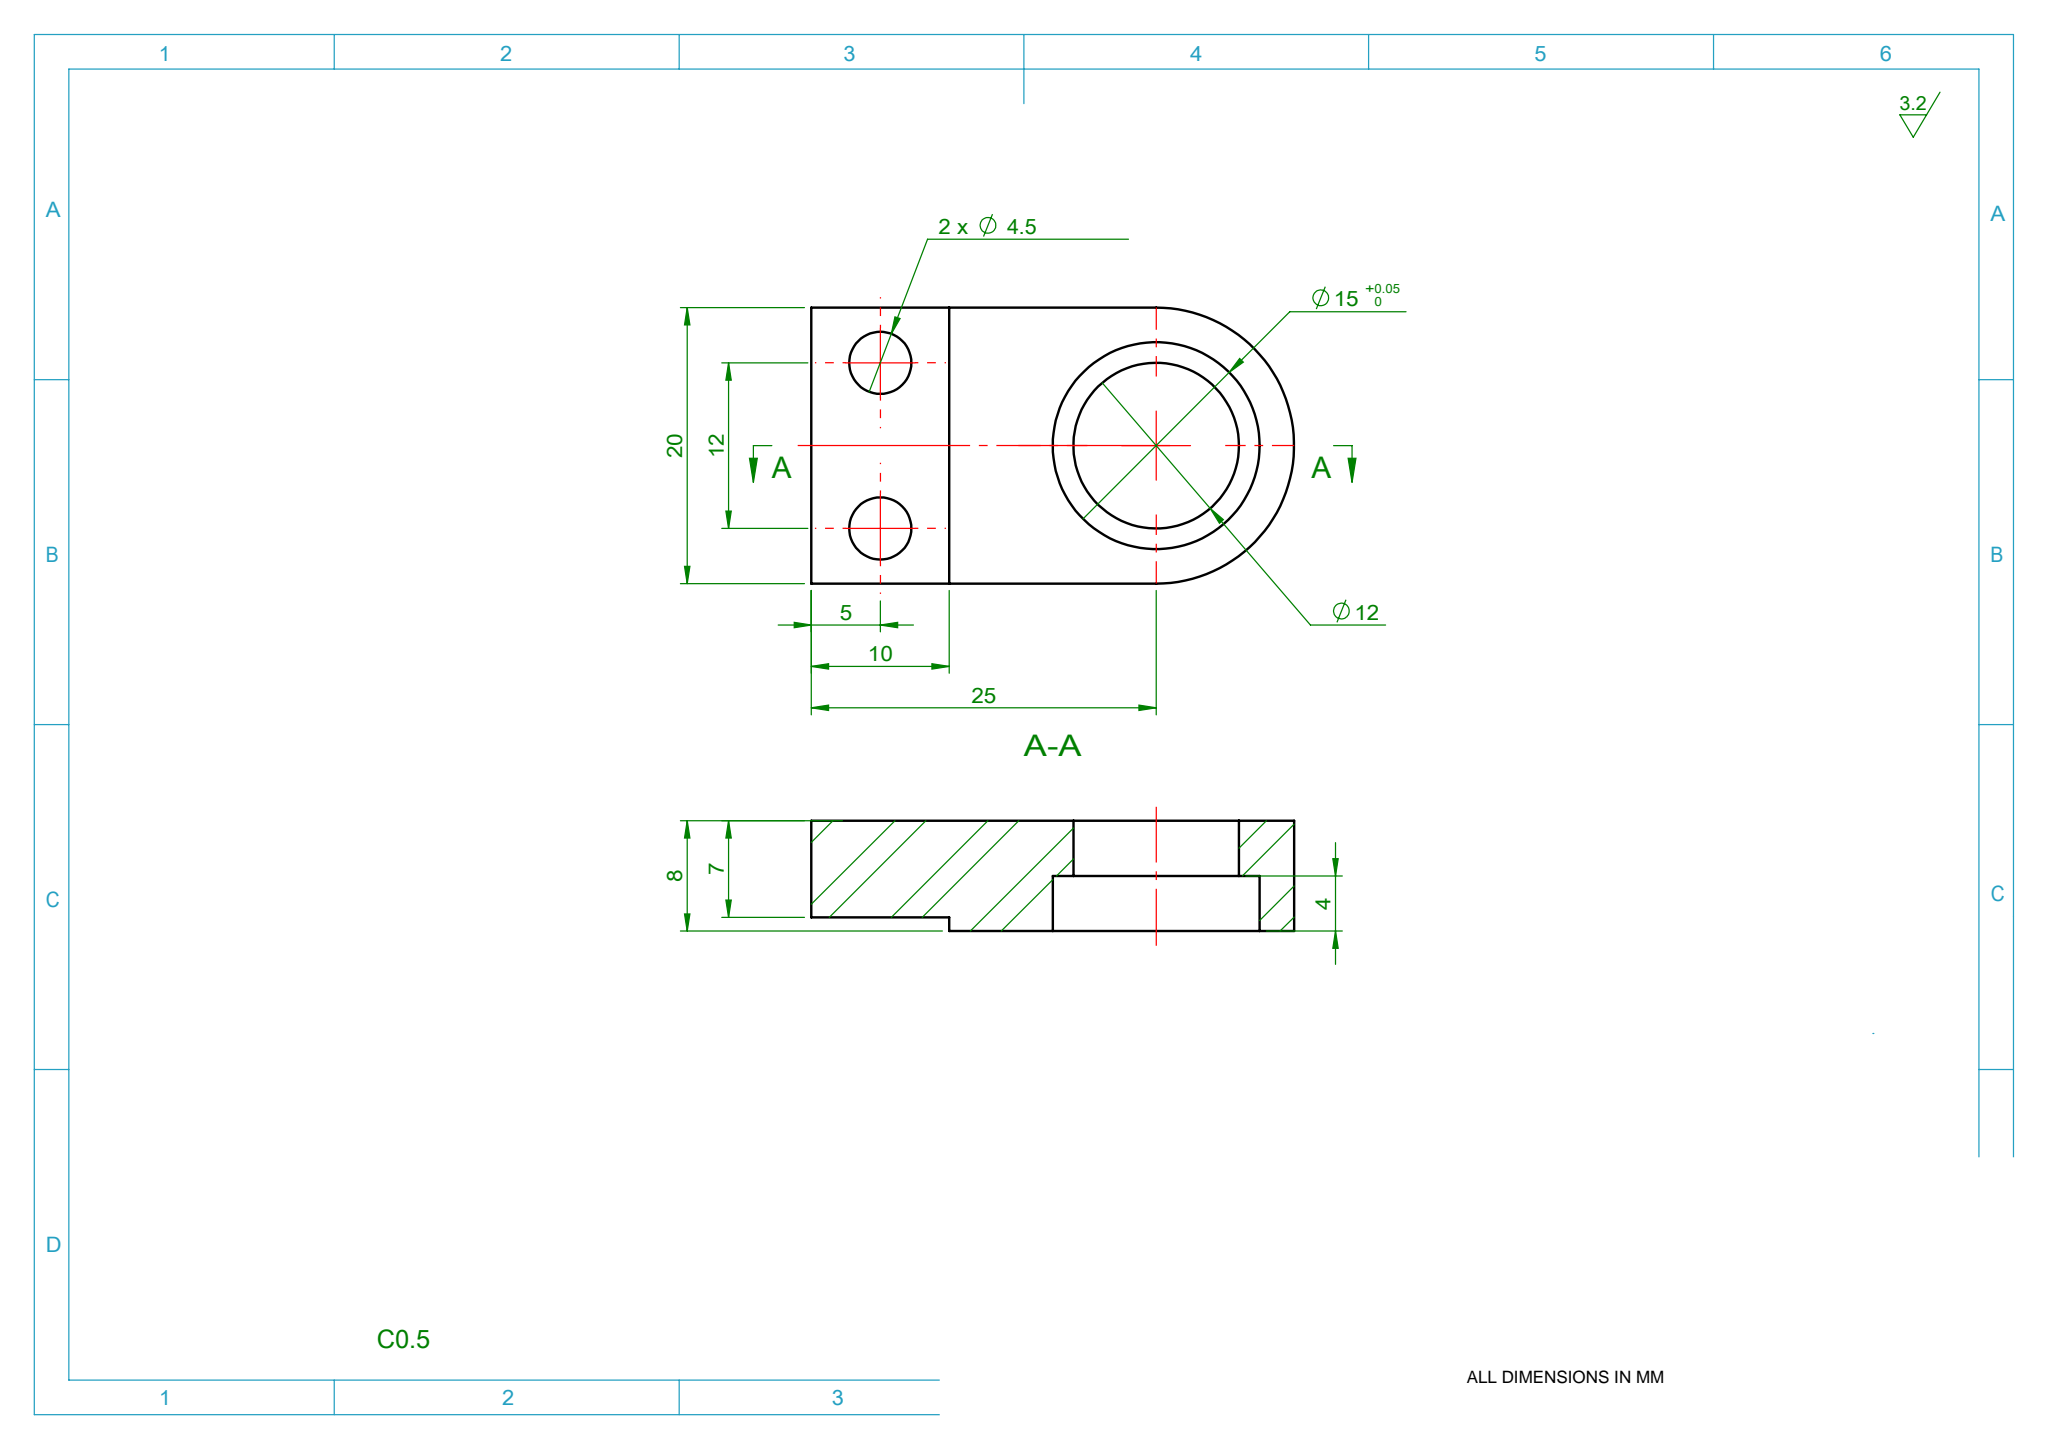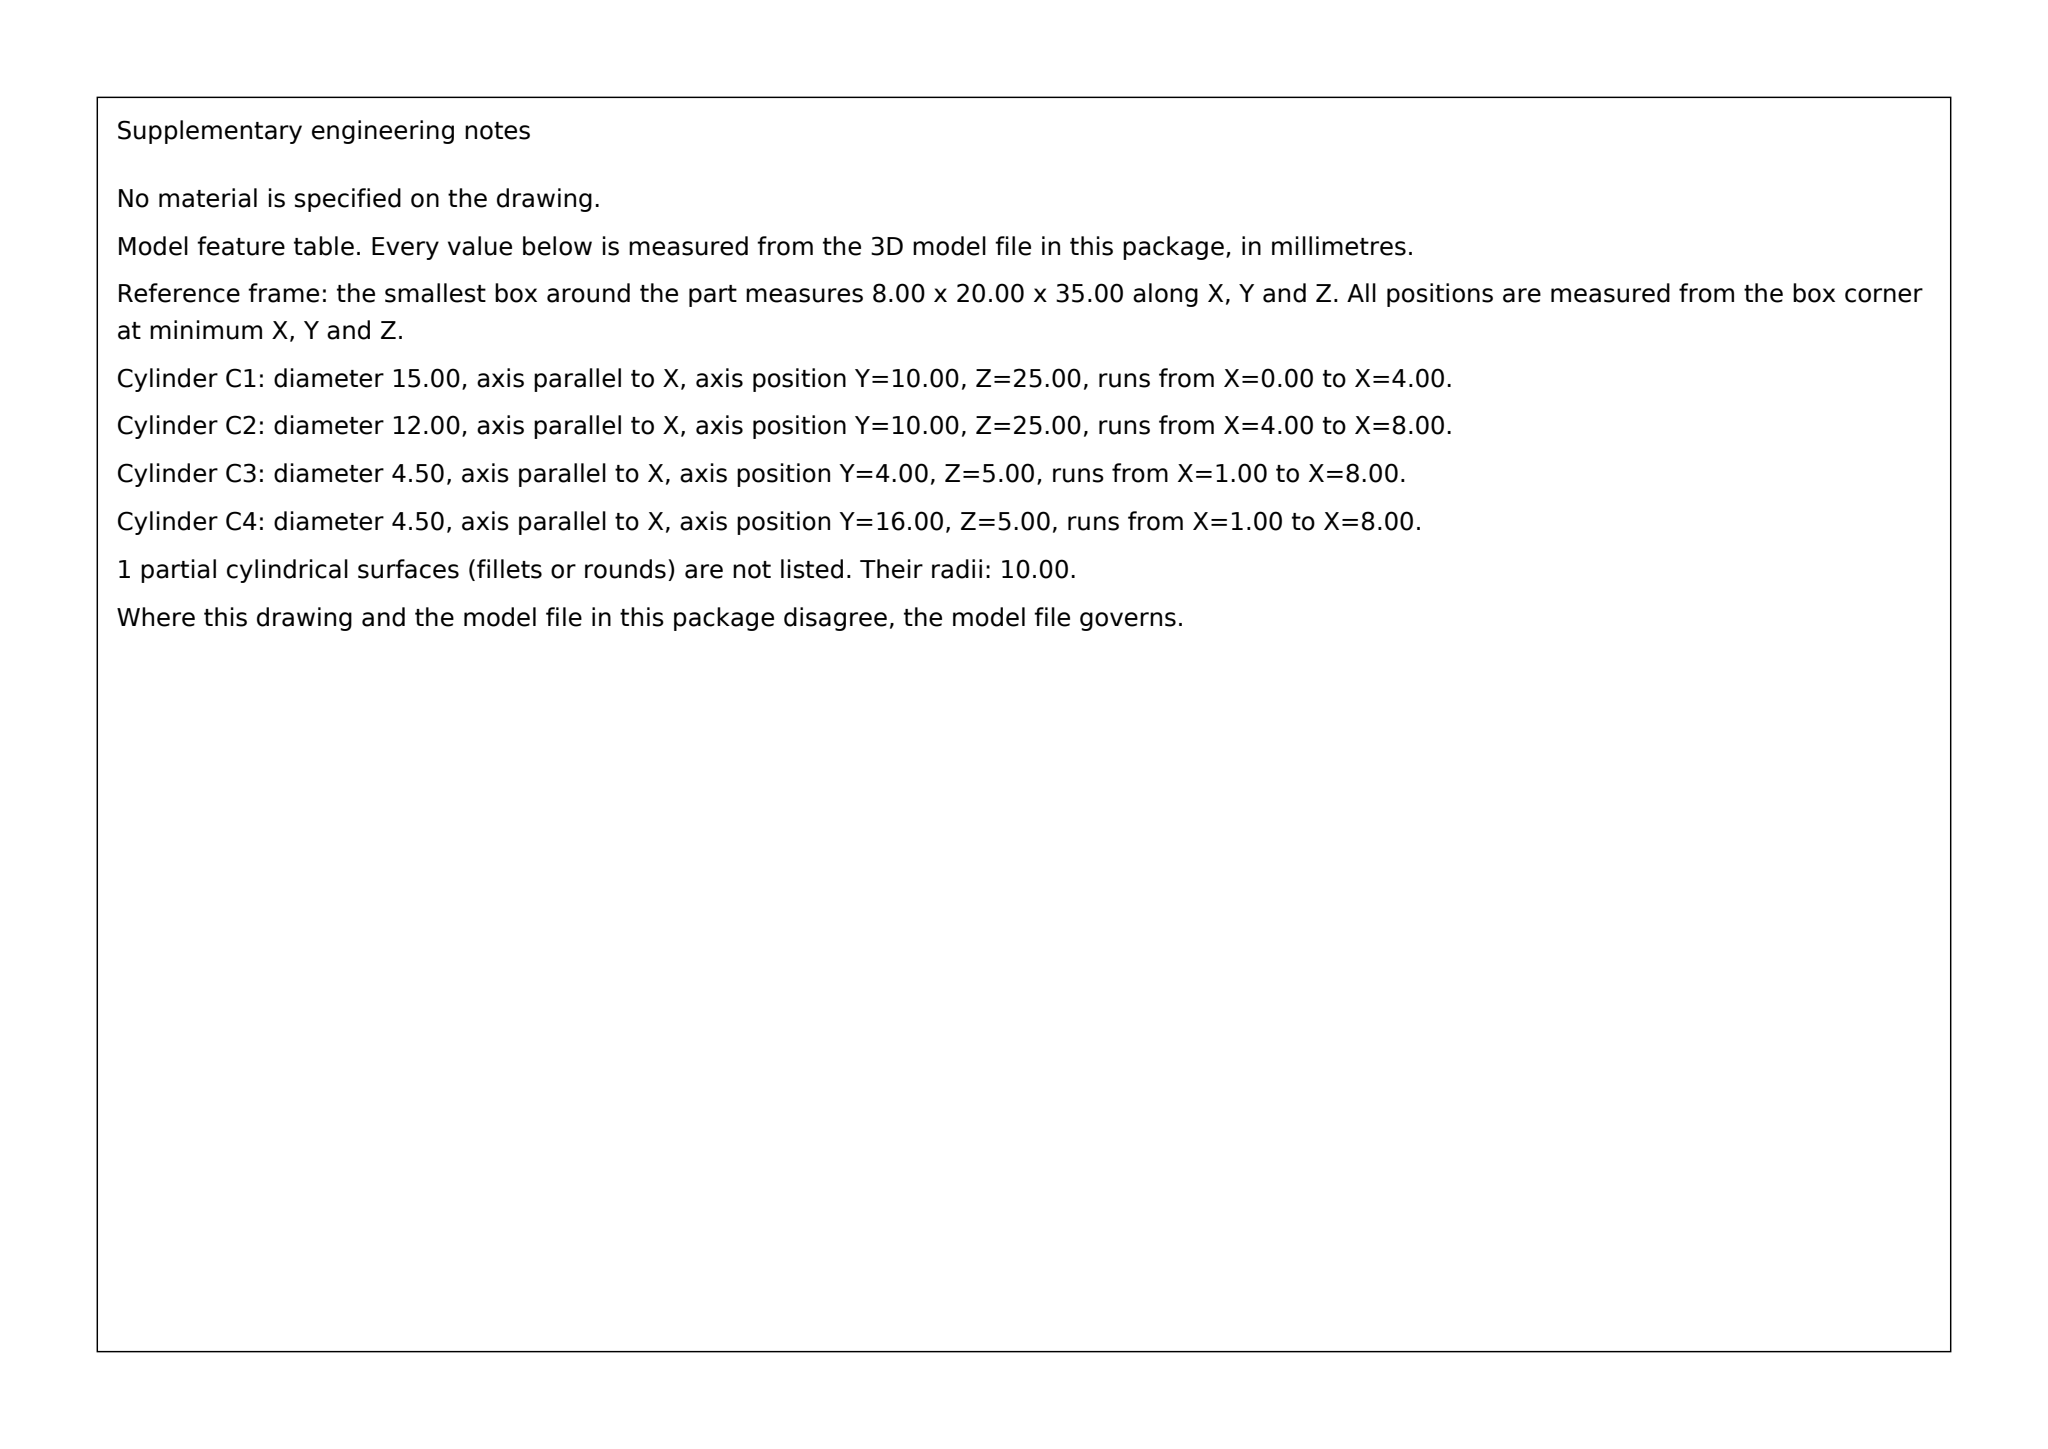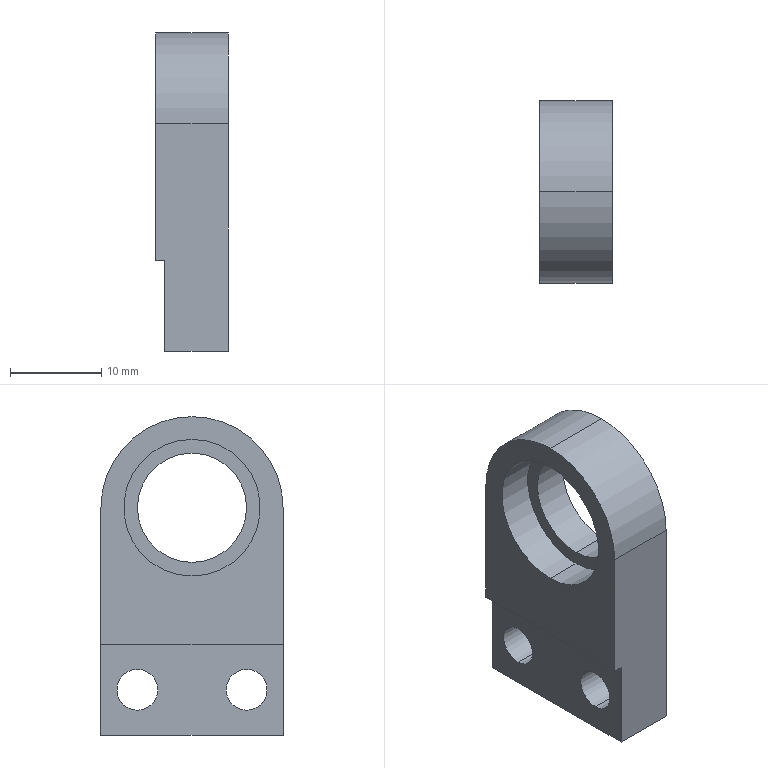Part | SolidWorks | mm | 1 solid | 18 faces | box 8 x 20 x 35 mm | volume 3675 mm3 | cylinder 10 | plane 8 | commonest cylinder face diameters 4.5 x4 12 x2 15 x2 20 x2
build123d program:
from build123d import *

# Parameters (mm, degrees)
BOSS_EXTRUDE1_DEPTH  = 8
SKETCH2_R            = 7.5
CUT_EXTRUDE1_DEPTH   = 4
SKETCH3_R            = 6
CUT_EXTRUDE2_DEPTH   = 28.221
SKETCH4_W            = 10
SKETCH4_H            = 20
CUT_EXTRUDE3_DEPTH   = 1
M4_CLEARANCE_HOLE1_D = 4.5


with BuildPart() as part:
    # Sketch1 → Boss-Extrude1 (new body)
    with BuildSketch(Plane(origin=(0, 0, 0), x_dir=(0, 0, -1), z_dir=(1, 0, 0))):
        with BuildLine():
            Line((0, 10), (25, 10))
            Line((25, 10), (25, -10))
            Line((25, -10), (0, -10))
            ThreePointArc((0, -10), (-10, 0), (0, 10))
        make_face()
    extrude(amount=BOSS_EXTRUDE1_DEPTH)

    # Sketch2 → Cut-Extrude1 (cut)
    with BuildSketch(Plane.ZY):
        Circle(SKETCH2_R)
    extrude(amount=-CUT_EXTRUDE1_DEPTH, mode=Mode.SUBTRACT)

    # Sketch3 → Cut-Extrude2 (cut, through all)
    with BuildSketch(Plane.ZY.offset(-4)):
        Circle(SKETCH3_R)
    extrude(amount=-CUT_EXTRUDE2_DEPTH, mode=Mode.SUBTRACT)

    # Sketch4 → Cut-Extrude3 (cut)
    with BuildSketch(Plane.ZY):
        with Locations((-20, 0)):
            Rectangle(SKETCH4_W, SKETCH4_H)
    extrude(amount=-CUT_EXTRUDE3_DEPTH, mode=Mode.SUBTRACT)

    # M4 Clearance Hole1 (through all)
    with Locations(Plane(origin=(8, 0, 0), x_dir=(0, 0, -1), z_dir=(1, 0, 0))):
        with Locations((20, 6), (20, -6)):
            Hole(M4_CLEARANCE_HOLE1_D / 2)


solid = part.part
STEP:
#1=CARTESIAN_POINT('',(1.,6.,-22.25));
#2=VERTEX_POINT('',#1);
#3=CARTESIAN_POINT('',(1.,6.,-17.75));
#4=VERTEX_POINT('',#3);
#5=CARTESIAN_POINT('',(1.,6.,-20.));
#6=DIRECTION('',(-1.,0.,0.));
#7=DIRECTION('',(0.,0.,1.));
#8=AXIS2_PLACEMENT_3D('',#5,#6,#7);
#9=CIRCLE('',#8,2.25);
#10=EDGE_CURVE('',#2,#4,#9,.T.);
#11=ORIENTED_EDGE('',*,*,#10,.T.);
#12=CARTESIAN_POINT('',(8.,6.,-17.75));
#13=VERTEX_POINT('',#12);
#14=CARTESIAN_POINT('',(8.,6.,-17.75));
#15=DIRECTION('',(1.,0.,0.));
#16=VECTOR('',#15,1000.);
#17=LINE('',#14,#16);
#18=EDGE_CURVE('',#4,#13,#17,.T.);
#19=ORIENTED_EDGE('',*,*,#18,.T.);
#20=CARTESIAN_POINT('',(8.,6.,-22.25));
#21=VERTEX_POINT('',#20);
#22=CARTESIAN_POINT('',(8.,6.,-20.));
#23=DIRECTION('',(1.,0.,0.));
#24=DIRECTION('',(0.,0.,-1.));
#25=AXIS2_PLACEMENT_3D('',#22,#23,#24);
#26=CIRCLE('',#25,2.25);
#27=EDGE_CURVE('',#13,#21,#26,.T.);
#28=ORIENTED_EDGE('',*,*,#27,.T.);
#29=CARTESIAN_POINT('',(8.,6.,-22.25));
#30=DIRECTION('',(1.,0.,0.));
#31=VECTOR('',#30,1000.);
#32=LINE('',#29,#31);
#33=EDGE_CURVE('',#2,#21,#32,.T.);
#34=ORIENTED_EDGE('',*,*,#33,.F.);
#35=EDGE_LOOP('',(#11,#19,#28,#34));
#36=FACE_OUTER_BOUND('',#35,.T.);
#37=CARTESIAN_POINT('',(8.,6.,-20.));
#38=DIRECTION('',(1.,0.,0.));
#39=DIRECTION('',(0.,0.,-1.));
#40=AXIS2_PLACEMENT_3D('',#37,#38,#39);
#41=CYLINDRICAL_SURFACE('',#40,2.25);
#42=ADVANCED_FACE('',(#36),#41,.F.);
#43=CARTESIAN_POINT('',(1.,-6.,-22.25));
#44=VERTEX_POINT('',#43);
#45=CARTESIAN_POINT('',(1.,-6.,-17.75));
#46=VERTEX_POINT('',#45);
#47=CARTESIAN_POINT('',(1.,-6.,-20.));
#48=DIRECTION('',(-1.,0.,0.));
#49=DIRECTION('',(0.,0.,1.));
#50=AXIS2_PLACEMENT_3D('',#47,#48,#49);
#51=CIRCLE('',#50,2.25);
#52=EDGE_CURVE('',#44,#46,#51,.T.);
#53=ORIENTED_EDGE('',*,*,#52,.T.);
#54=CARTESIAN_POINT('',(8.,-6.,-17.75));
#55=VERTEX_POINT('',#54);
#56=CARTESIAN_POINT('',(8.,-6.,-17.75));
#57=DIRECTION('',(1.,0.,0.));
#58=VECTOR('',#57,1000.);
#59=LINE('',#56,#58);
#60=EDGE_CURVE('',#46,#55,#59,.T.);
#61=ORIENTED_EDGE('',*,*,#60,.T.);
#62=CARTESIAN_POINT('',(8.,-6.,-22.25));
#63=VERTEX_POINT('',#62);
#64=CARTESIAN_POINT('',(8.,-6.,-20.));
#65=DIRECTION('',(1.,0.,0.));
#66=DIRECTION('',(0.,0.,-1.));
#67=AXIS2_PLACEMENT_3D('',#64,#65,#66);
#68=CIRCLE('',#67,2.25);
#69=EDGE_CURVE('',#55,#63,#68,.T.);
#70=ORIENTED_EDGE('',*,*,#69,.T.);
#71=CARTESIAN_POINT('',(8.,-6.,-22.25));
#72=DIRECTION('',(1.,0.,0.));
#73=VECTOR('',#72,1000.);
#74=LINE('',#71,#73);
#75=EDGE_CURVE('',#44,#63,#74,.T.);
#76=ORIENTED_EDGE('',*,*,#75,.F.);
#77=EDGE_LOOP('',(#53,#61,#70,#76));
#78=FACE_OUTER_BOUND('',#77,.T.);
#79=CARTESIAN_POINT('',(8.,-6.,-20.));
#80=DIRECTION('',(1.,0.,0.));
#81=DIRECTION('',(0.,0.,-1.));
#82=AXIS2_PLACEMENT_3D('',#79,#80,#81);
#83=CYLINDRICAL_SURFACE('',#82,2.25);
#84=ADVANCED_FACE('',(#78),#83,.F.);
#85=CARTESIAN_POINT('',(8.,0.,-6.));
#86=VERTEX_POINT('',#85);
#87=CARTESIAN_POINT('',(8.,0.,6.));
#88=VERTEX_POINT('',#87);
#89=CARTESIAN_POINT('',(8.,0.,0.));
#90=DIRECTION('',(-1.,0.,0.));
#91=DIRECTION('',(0.,0.,1.));
#92=AXIS2_PLACEMENT_3D('',#89,#90,#91);
#93=CIRCLE('',#92,6.);
#94=EDGE_CURVE('',#86,#88,#93,.T.);
#95=ORIENTED_EDGE('',*,*,#94,.F.);
#96=CARTESIAN_POINT('',(4.,0.,-6.));
#97=VERTEX_POINT('',#96);
#98=CARTESIAN_POINT('',(8.,0.,-6.));
#99=DIRECTION('',(-1.,0.,0.));
#100=VECTOR('',#99,1000.);
#101=LINE('',#98,#100);
#102=EDGE_CURVE('',#86,#97,#101,.T.);
#103=ORIENTED_EDGE('',*,*,#102,.T.);
#104=CARTESIAN_POINT('',(4.,0.,6.));
#105=VERTEX_POINT('',#104);
#106=CARTESIAN_POINT('',(4.,0.,0.));
#107=DIRECTION('',(-1.,0.,0.));
#108=DIRECTION('',(0.,0.,1.));
#109=AXIS2_PLACEMENT_3D('',#106,#107,#108);
#110=CIRCLE('',#109,6.);
#111=EDGE_CURVE('',#97,#105,#110,.T.);
#112=ORIENTED_EDGE('',*,*,#111,.T.);
#113=CARTESIAN_POINT('',(8.,0.,6.));
#114=DIRECTION('',(-1.,0.,0.));
#115=VECTOR('',#114,1000.);
#116=LINE('',#113,#115);
#117=EDGE_CURVE('',#88,#105,#116,.T.);
#118=ORIENTED_EDGE('',*,*,#117,.F.);
#119=EDGE_LOOP('',(#95,#103,#112,#118));
#120=FACE_OUTER_BOUND('',#119,.T.);
#121=CARTESIAN_POINT('',(8.,0.,0.));
#122=DIRECTION('',(-1.,0.,0.));
#123=DIRECTION('',(0.,0.,1.));
#124=AXIS2_PLACEMENT_3D('',#121,#122,#123);
#125=CYLINDRICAL_SURFACE('',#124,6.);
#126=ADVANCED_FACE('',(#120),#125,.F.);
#127=CARTESIAN_POINT('',(4.,0.,-7.5));
#128=VERTEX_POINT('',#127);
#129=CARTESIAN_POINT('',(4.,0.,7.5));
#130=VERTEX_POINT('',#129);
#131=CARTESIAN_POINT('',(4.,0.,0.));
#132=DIRECTION('',(-1.,0.,0.));
#133=DIRECTION('',(0.,0.,1.));
#134=AXIS2_PLACEMENT_3D('',#131,#132,#133);
#135=CIRCLE('',#134,7.5);
#136=EDGE_CURVE('',#128,#130,#135,.T.);
#137=ORIENTED_EDGE('',*,*,#136,.F.);
#138=CARTESIAN_POINT('',(0.,0.,-7.5));
#139=VERTEX_POINT('',#138);
#140=CARTESIAN_POINT('',(4.,0.,-7.5));
#141=DIRECTION('',(-1.,0.,0.));
#142=VECTOR('',#141,1000.);
#143=LINE('',#140,#142);
#144=EDGE_CURVE('',#128,#139,#143,.T.);
#145=ORIENTED_EDGE('',*,*,#144,.T.);
#146=CARTESIAN_POINT('',(0.,0.,7.5));
#147=VERTEX_POINT('',#146);
#148=CARTESIAN_POINT('',(0.,0.,0.));
#149=DIRECTION('',(-1.,0.,0.));
#150=DIRECTION('',(0.,0.,1.));
#151=AXIS2_PLACEMENT_3D('',#148,#149,#150);
#152=CIRCLE('',#151,7.5);
#153=EDGE_CURVE('',#139,#147,#152,.T.);
#154=ORIENTED_EDGE('',*,*,#153,.T.);
#155=CARTESIAN_POINT('',(4.,0.,7.5));
#156=DIRECTION('',(-1.,0.,0.));
#157=VECTOR('',#156,1000.);
#158=LINE('',#155,#157);
#159=EDGE_CURVE('',#130,#147,#158,.T.);
#160=ORIENTED_EDGE('',*,*,#159,.F.);
#161=EDGE_LOOP('',(#137,#145,#154,#160));
#162=FACE_OUTER_BOUND('',#161,.T.);
#163=CARTESIAN_POINT('',(4.,0.,0.));
#164=DIRECTION('',(-1.,0.,0.));
#165=DIRECTION('',(0.,0.,1.));
#166=AXIS2_PLACEMENT_3D('',#163,#164,#165);
#167=CYLINDRICAL_SURFACE('',#166,7.5);
#168=ADVANCED_FACE('',(#162),#167,.F.);
#169=CARTESIAN_POINT('',(8.,0.,10.));
#170=VERTEX_POINT('',#169);
#171=CARTESIAN_POINT('',(8.,-10.,0.));
#172=VERTEX_POINT('',#171);
#173=CARTESIAN_POINT('',(8.,0.,0.));
#174=DIRECTION('',(1.,0.,0.));
#175=DIRECTION('',(0.,0.,-1.));
#176=AXIS2_PLACEMENT_3D('',#173,#174,#175);
#177=CIRCLE('',#176,10.);
#178=EDGE_CURVE('',#170,#172,#177,.T.);
#179=ORIENTED_EDGE('',*,*,#178,.F.);
#180=CARTESIAN_POINT('',(0.,0.,10.));
#181=VERTEX_POINT('',#180);
#182=CARTESIAN_POINT('',(8.,0.,10.));
#183=DIRECTION('',(-1.,0.,0.));
#184=VECTOR('',#183,1000.);
#185=LINE('',#182,#184);
#186=EDGE_CURVE('',#170,#181,#185,.T.);
#187=ORIENTED_EDGE('',*,*,#186,.T.);
#188=CARTESIAN_POINT('',(0.,-10.,0.));
#189=VERTEX_POINT('',#188);
#190=CARTESIAN_POINT('',(0.,0.,0.));
#191=DIRECTION('',(1.,0.,0.));
#192=DIRECTION('',(0.,0.,-1.));
#193=AXIS2_PLACEMENT_3D('',#190,#191,#192);
#194=CIRCLE('',#193,10.);
#195=EDGE_CURVE('',#181,#189,#194,.T.);
#196=ORIENTED_EDGE('',*,*,#195,.T.);
#197=CARTESIAN_POINT('',(8.,-10.,0.));
#198=DIRECTION('',(-1.,0.,0.));
#199=VECTOR('',#198,1000.);
#200=LINE('',#197,#199);
#201=EDGE_CURVE('',#172,#189,#200,.T.);
#202=ORIENTED_EDGE('',*,*,#201,.F.);
#203=EDGE_LOOP('',(#179,#187,#196,#202));
#204=FACE_OUTER_BOUND('',#203,.T.);
#205=CARTESIAN_POINT('',(8.,0.,0.));
#206=DIRECTION('',(-1.,0.,0.));
#207=DIRECTION('',(0.,0.,1.));
#208=AXIS2_PLACEMENT_3D('',#205,#206,#207);
#209=CYLINDRICAL_SURFACE('',#208,10.);
#210=ADVANCED_FACE('',(#204),#209,.T.);
#211=CARTESIAN_POINT('',(1.,10.,-25.));
#212=VERTEX_POINT('',#211);
#213=CARTESIAN_POINT('',(1.,-10.,-25.));
#214=VERTEX_POINT('',#213);
#215=CARTESIAN_POINT('',(1.,-10.,-25.));
#216=DIRECTION('',(0.,-1.,0.));
#217=VECTOR('',#216,1000.);
#218=LINE('',#215,#217);
#219=EDGE_CURVE('',#212,#214,#218,.T.);
#220=ORIENTED_EDGE('',*,*,#219,.F.);
#221=CARTESIAN_POINT('',(8.,10.,-25.));
#222=VERTEX_POINT('',#221);
#223=CARTESIAN_POINT('',(8.,10.,-25.));
#224=DIRECTION('',(-1.,0.,0.));
#225=VECTOR('',#224,1000.);
#226=LINE('',#223,#225);
#227=EDGE_CURVE('',#222,#212,#226,.T.);
#228=ORIENTED_EDGE('',*,*,#227,.F.);
#229=CARTESIAN_POINT('',(8.,-10.,-25.));
#230=VERTEX_POINT('',#229);
#231=CARTESIAN_POINT('',(8.,10.,-25.));
#232=DIRECTION('',(0.,1.,0.));
#233=VECTOR('',#232,1000.);
#234=LINE('',#231,#233);
#235=EDGE_CURVE('',#230,#222,#234,.T.);
#236=ORIENTED_EDGE('',*,*,#235,.F.);
#237=CARTESIAN_POINT('',(8.,-10.,-25.));
#238=DIRECTION('',(-1.,0.,0.));
#239=VECTOR('',#238,1000.);
#240=LINE('',#237,#239);
#241=EDGE_CURVE('',#230,#214,#240,.T.);
#242=ORIENTED_EDGE('',*,*,#241,.T.);
#243=EDGE_LOOP('',(#220,#228,#236,#242));
#244=FACE_OUTER_BOUND('',#243,.T.);
#245=CARTESIAN_POINT('',(8.,10.,-25.));
#246=DIRECTION('',(0.,0.,1.));
#247=DIRECTION('',(1.,0.,0.));
#248=AXIS2_PLACEMENT_3D('',#245,#246,#247);
#249=PLANE('',#248);
#250=ADVANCED_FACE('',(#244),#249,.F.);
#251=ORIENTED_EDGE('',*,*,#186,.F.);
#252=CARTESIAN_POINT('',(8.,10.,0.));
#253=VERTEX_POINT('',#252);
#254=CARTESIAN_POINT('',(8.,0.,0.));
#255=DIRECTION('',(1.,0.,0.));
#256=DIRECTION('',(0.,0.,-1.));
#257=AXIS2_PLACEMENT_3D('',#254,#255,#256);
#258=CIRCLE('',#257,10.);
#259=EDGE_CURVE('',#253,#170,#258,.T.);
#260=ORIENTED_EDGE('',*,*,#259,.F.);
#261=CARTESIAN_POINT('',(0.,10.,0.));
#262=VERTEX_POINT('',#261);
#263=CARTESIAN_POINT('',(8.,10.,0.));
#264=DIRECTION('',(-1.,0.,0.));
#265=VECTOR('',#264,1000.);
#266=LINE('',#263,#265);
#267=EDGE_CURVE('',#253,#262,#266,.T.);
#268=ORIENTED_EDGE('',*,*,#267,.T.);
#269=CARTESIAN_POINT('',(0.,0.,0.));
#270=DIRECTION('',(1.,0.,0.));
#271=DIRECTION('',(0.,0.,-1.));
#272=AXIS2_PLACEMENT_3D('',#269,#270,#271);
#273=CIRCLE('',#272,10.);
#274=EDGE_CURVE('',#262,#181,#273,.T.);
#275=ORIENTED_EDGE('',*,*,#274,.T.);
#276=EDGE_LOOP('',(#251,#260,#268,#275));
#277=FACE_OUTER_BOUND('',#276,.T.);
#278=CARTESIAN_POINT('',(8.,0.,0.));
#279=DIRECTION('',(-1.,0.,0.));
#280=DIRECTION('',(0.,0.,1.));
#281=AXIS2_PLACEMENT_3D('',#278,#279,#280);
#282=CYLINDRICAL_SURFACE('',#281,10.);
#283=ADVANCED_FACE('',(#277),#282,.T.);
#284=CARTESIAN_POINT('',(0.,-10.,-15.));
#285=VERTEX_POINT('',#284);
#286=CARTESIAN_POINT('',(0.,-10.,0.));
#287=DIRECTION('',(0.,0.,-1.));
#288=VECTOR('',#287,1000.);
#289=LINE('',#286,#288);
#290=EDGE_CURVE('',#189,#285,#289,.T.);
#291=ORIENTED_EDGE('',*,*,#290,.T.);
#292=CARTESIAN_POINT('',(1.,-10.,-15.));
#293=VERTEX_POINT('',#292);
#294=CARTESIAN_POINT('',(1.,-10.,-15.));
#295=DIRECTION('',(-1.,0.,0.));
#296=VECTOR('',#295,1000.);
#297=LINE('',#294,#296);
#298=EDGE_CURVE('',#293,#285,#297,.T.);
#299=ORIENTED_EDGE('',*,*,#298,.F.);
#300=CARTESIAN_POINT('',(1.,-10.,-15.));
#301=DIRECTION('',(0.,0.,1.));
#302=VECTOR('',#301,1000.);
#303=LINE('',#300,#302);
#304=EDGE_CURVE('',#214,#293,#303,.T.);
#305=ORIENTED_EDGE('',*,*,#304,.F.);
#306=ORIENTED_EDGE('',*,*,#241,.F.);
#307=CARTESIAN_POINT('',(8.,-10.,0.));
#308=DIRECTION('',(0.,0.,-1.));
#309=VECTOR('',#308,1000.);
#310=LINE('',#307,#309);
#311=EDGE_CURVE('',#172,#230,#310,.T.);
#312=ORIENTED_EDGE('',*,*,#311,.F.);
#313=ORIENTED_EDGE('',*,*,#201,.T.);
#314=EDGE_LOOP('',(#291,#299,#305,#306,#312,#313));
#315=FACE_OUTER_BOUND('',#314,.T.);
#316=CARTESIAN_POINT('',(8.,-10.,0.));
#317=DIRECTION('',(0.,1.,0.));
#318=DIRECTION('',(0.,0.,1.));
#319=AXIS2_PLACEMENT_3D('',#316,#317,#318);
#320=PLANE('',#319);
#321=ADVANCED_FACE('',(#315),#320,.F.);
#322=CARTESIAN_POINT('',(1.,10.,-15.));
#323=VERTEX_POINT('',#322);
#324=CARTESIAN_POINT('',(1.,10.,-15.));
#325=DIRECTION('',(0.,0.,-1.));
#326=VECTOR('',#325,1000.);
#327=LINE('',#324,#326);
#328=EDGE_CURVE('',#323,#212,#327,.T.);
#329=ORIENTED_EDGE('',*,*,#328,.F.);
#330=CARTESIAN_POINT('',(0.,10.,-15.));
#331=VERTEX_POINT('',#330);
#332=CARTESIAN_POINT('',(1.,10.,-15.));
#333=DIRECTION('',(-1.,0.,0.));
#334=VECTOR('',#333,1000.);
#335=LINE('',#332,#334);
#336=EDGE_CURVE('',#323,#331,#335,.T.);
#337=ORIENTED_EDGE('',*,*,#336,.T.);
#338=CARTESIAN_POINT('',(0.,10.,0.));
#339=DIRECTION('',(0.,0.,1.));
#340=VECTOR('',#339,1000.);
#341=LINE('',#338,#340);
#342=EDGE_CURVE('',#331,#262,#341,.T.);
#343=ORIENTED_EDGE('',*,*,#342,.T.);
#344=ORIENTED_EDGE('',*,*,#267,.F.);
#345=CARTESIAN_POINT('',(8.,10.,0.));
#346=DIRECTION('',(0.,0.,1.));
#347=VECTOR('',#346,1000.);
#348=LINE('',#345,#347);
#349=EDGE_CURVE('',#222,#253,#348,.T.);
#350=ORIENTED_EDGE('',*,*,#349,.F.);
#351=ORIENTED_EDGE('',*,*,#227,.T.);
#352=EDGE_LOOP('',(#329,#337,#343,#344,#350,#351));
#353=FACE_OUTER_BOUND('',#352,.T.);
#354=CARTESIAN_POINT('',(8.,10.,0.));
#355=DIRECTION('',(0.,-1.,0.));
#356=DIRECTION('',(0.,0.,-1.));
#357=AXIS2_PLACEMENT_3D('',#354,#355,#356);
#358=PLANE('',#357);
#359=ADVANCED_FACE('',(#353),#358,.F.);
#360=CARTESIAN_POINT('',(8.,6.,-20.));
#361=DIRECTION('',(1.,0.,0.));
#362=DIRECTION('',(0.,0.,-1.));
#363=AXIS2_PLACEMENT_3D('',#360,#361,#362);
#364=CIRCLE('',#363,2.25);
#365=EDGE_CURVE('',#21,#13,#364,.T.);
#366=ORIENTED_EDGE('',*,*,#365,.F.);
#367=ORIENTED_EDGE('',*,*,#27,.F.);
#368=EDGE_LOOP('',(#366,#367));
#369=FACE_BOUND('',#368,.T.);
#370=CARTESIAN_POINT('',(8.,-6.,-20.));
#371=DIRECTION('',(1.,0.,0.));
#372=DIRECTION('',(0.,0.,-1.));
#373=AXIS2_PLACEMENT_3D('',#370,#371,#372);
#374=CIRCLE('',#373,2.25);
#375=EDGE_CURVE('',#63,#55,#374,.T.);
#376=ORIENTED_EDGE('',*,*,#375,.F.);
#377=ORIENTED_EDGE('',*,*,#69,.F.);
#378=EDGE_LOOP('',(#376,#377));
#379=FACE_BOUND('',#378,.T.);
#380=CARTESIAN_POINT('',(8.,0.,0.));
#381=DIRECTION('',(-1.,0.,0.));
#382=DIRECTION('',(0.,0.,1.));
#383=AXIS2_PLACEMENT_3D('',#380,#381,#382);
#384=CIRCLE('',#383,6.);
#385=EDGE_CURVE('',#88,#86,#384,.T.);
#386=ORIENTED_EDGE('',*,*,#385,.T.);
#387=ORIENTED_EDGE('',*,*,#94,.T.);
#388=EDGE_LOOP('',(#386,#387));
#389=FACE_BOUND('',#388,.T.);
#390=ORIENTED_EDGE('',*,*,#259,.T.);
#391=ORIENTED_EDGE('',*,*,#178,.T.);
#392=ORIENTED_EDGE('',*,*,#311,.T.);
#393=ORIENTED_EDGE('',*,*,#235,.T.);
#394=ORIENTED_EDGE('',*,*,#349,.T.);
#395=EDGE_LOOP('',(#390,#391,#392,#393,#394));
#396=FACE_OUTER_BOUND('',#395,.T.);
#397=CARTESIAN_POINT('',(8.,0.,0.));
#398=DIRECTION('',(1.,0.,0.));
#399=DIRECTION('',(0.,0.,-1.));
#400=AXIS2_PLACEMENT_3D('',#397,#398,#399);
#401=PLANE('',#400);
#402=ADVANCED_FACE('',(#369,#379,#389,#396),#401,.T.);
#403=CARTESIAN_POINT('',(0.,0.,0.));
#404=DIRECTION('',(-1.,0.,0.));
#405=DIRECTION('',(0.,0.,1.));
#406=AXIS2_PLACEMENT_3D('',#403,#404,#405);
#407=CIRCLE('',#406,7.5);
#408=EDGE_CURVE('',#147,#139,#407,.T.);
#409=ORIENTED_EDGE('',*,*,#408,.F.);
#410=ORIENTED_EDGE('',*,*,#153,.F.);
#411=EDGE_LOOP('',(#409,#410));
#412=FACE_BOUND('',#411,.T.);
#413=ORIENTED_EDGE('',*,*,#342,.F.);
#414=CARTESIAN_POINT('',(0.,-10.,-15.));
#415=DIRECTION('',(0.,1.,0.));
#416=VECTOR('',#415,1000.);
#417=LINE('',#414,#416);
#418=EDGE_CURVE('',#285,#331,#417,.T.);
#419=ORIENTED_EDGE('',*,*,#418,.F.);
#420=ORIENTED_EDGE('',*,*,#290,.F.);
#421=ORIENTED_EDGE('',*,*,#195,.F.);
#422=ORIENTED_EDGE('',*,*,#274,.F.);
#423=EDGE_LOOP('',(#413,#419,#420,#421,#422));
#424=FACE_OUTER_BOUND('',#423,.T.);
#425=CARTESIAN_POINT('',(0.,0.,0.));
#426=DIRECTION('',(1.,0.,0.));
#427=DIRECTION('',(0.,0.,-1.));
#428=AXIS2_PLACEMENT_3D('',#425,#426,#427);
#429=PLANE('',#428);
#430=ADVANCED_FACE('',(#412,#424),#429,.F.);
#431=ORIENTED_EDGE('',*,*,#144,.F.);
#432=CARTESIAN_POINT('',(4.,0.,0.));
#433=DIRECTION('',(-1.,0.,0.));
#434=DIRECTION('',(0.,0.,1.));
#435=AXIS2_PLACEMENT_3D('',#432,#433,#434);
#436=CIRCLE('',#435,7.5);
#437=EDGE_CURVE('',#130,#128,#436,.T.);
#438=ORIENTED_EDGE('',*,*,#437,.F.);
#439=ORIENTED_EDGE('',*,*,#159,.T.);
#440=ORIENTED_EDGE('',*,*,#408,.T.);
#441=EDGE_LOOP('',(#431,#438,#439,#440));
#442=FACE_OUTER_BOUND('',#441,.T.);
#443=CARTESIAN_POINT('',(4.,0.,0.));
#444=DIRECTION('',(-1.,0.,0.));
#445=DIRECTION('',(0.,0.,1.));
#446=AXIS2_PLACEMENT_3D('',#443,#444,#445);
#447=CYLINDRICAL_SURFACE('',#446,7.5);
#448=ADVANCED_FACE('',(#442),#447,.F.);
#449=CARTESIAN_POINT('',(4.,0.,0.));
#450=DIRECTION('',(-1.,0.,0.));
#451=DIRECTION('',(0.,0.,1.));
#452=AXIS2_PLACEMENT_3D('',#449,#450,#451);
#453=CIRCLE('',#452,6.);
#454=EDGE_CURVE('',#105,#97,#453,.T.);
#455=ORIENTED_EDGE('',*,*,#454,.F.);
#456=ORIENTED_EDGE('',*,*,#111,.F.);
#457=EDGE_LOOP('',(#455,#456));
#458=FACE_BOUND('',#457,.T.);
#459=ORIENTED_EDGE('',*,*,#437,.T.);
#460=ORIENTED_EDGE('',*,*,#136,.T.);
#461=EDGE_LOOP('',(#459,#460));
#462=FACE_OUTER_BOUND('',#461,.T.);
#463=CARTESIAN_POINT('',(4.,0.,0.));
#464=DIRECTION('',(-1.,0.,0.));
#465=DIRECTION('',(0.,0.,1.));
#466=AXIS2_PLACEMENT_3D('',#463,#464,#465);
#467=PLANE('',#466);
#468=ADVANCED_FACE('',(#458,#462),#467,.T.);
#469=ORIENTED_EDGE('',*,*,#102,.F.);
#470=ORIENTED_EDGE('',*,*,#385,.F.);
#471=ORIENTED_EDGE('',*,*,#117,.T.);
#472=ORIENTED_EDGE('',*,*,#454,.T.);
#473=EDGE_LOOP('',(#469,#470,#471,#472));
#474=FACE_OUTER_BOUND('',#473,.T.);
#475=CARTESIAN_POINT('',(8.,0.,0.));
#476=DIRECTION('',(-1.,0.,0.));
#477=DIRECTION('',(0.,0.,1.));
#478=AXIS2_PLACEMENT_3D('',#475,#476,#477);
#479=CYLINDRICAL_SURFACE('',#478,6.);
#480=ADVANCED_FACE('',(#474),#479,.F.);
#481=ORIENTED_EDGE('',*,*,#418,.T.);
#482=ORIENTED_EDGE('',*,*,#336,.F.);
#483=CARTESIAN_POINT('',(1.,-10.,-15.));
#484=DIRECTION('',(0.,1.,0.));
#485=VECTOR('',#484,1000.);
#486=LINE('',#483,#485);
#487=EDGE_CURVE('',#293,#323,#486,.T.);
#488=ORIENTED_EDGE('',*,*,#487,.F.);
#489=ORIENTED_EDGE('',*,*,#298,.T.);
#490=EDGE_LOOP('',(#481,#482,#488,#489));
#491=FACE_OUTER_BOUND('',#490,.T.);
#492=CARTESIAN_POINT('',(1.,-10.,-15.));
#493=DIRECTION('',(0.,-0.,1.));
#494=DIRECTION('',(0.,-1.,-0.));
#495=AXIS2_PLACEMENT_3D('',#492,#493,#494);
#496=PLANE('',#495);
#497=ADVANCED_FACE('',(#491),#496,.F.);
#498=ORIENTED_EDGE('',*,*,#10,.F.);
#499=CARTESIAN_POINT('',(1.,6.,-20.));
#500=DIRECTION('',(-1.,0.,0.));
#501=DIRECTION('',(0.,0.,1.));
#502=AXIS2_PLACEMENT_3D('',#499,#500,#501);
#503=CIRCLE('',#502,2.25);
#504=EDGE_CURVE('',#4,#2,#503,.T.);
#505=ORIENTED_EDGE('',*,*,#504,.F.);
#506=EDGE_LOOP('',(#498,#505));
#507=FACE_BOUND('',#506,.T.);
#508=ORIENTED_EDGE('',*,*,#52,.F.);
#509=CARTESIAN_POINT('',(1.,-6.,-20.));
#510=DIRECTION('',(-1.,0.,0.));
#511=DIRECTION('',(0.,0.,1.));
#512=AXIS2_PLACEMENT_3D('',#509,#510,#511);
#513=CIRCLE('',#512,2.25);
#514=EDGE_CURVE('',#46,#44,#513,.T.);
#515=ORIENTED_EDGE('',*,*,#514,.F.);
#516=EDGE_LOOP('',(#508,#515));
#517=FACE_BOUND('',#516,.T.);
#518=ORIENTED_EDGE('',*,*,#219,.T.);
#519=ORIENTED_EDGE('',*,*,#304,.T.);
#520=ORIENTED_EDGE('',*,*,#487,.T.);
#521=ORIENTED_EDGE('',*,*,#328,.T.);
#522=EDGE_LOOP('',(#518,#519,#520,#521));
#523=FACE_OUTER_BOUND('',#522,.T.);
#524=CARTESIAN_POINT('',(1.,0.,0.));
#525=DIRECTION('',(-1.,0.,0.));
#526=DIRECTION('',(0.,0.,1.));
#527=AXIS2_PLACEMENT_3D('',#524,#525,#526);
#528=PLANE('',#527);
#529=ADVANCED_FACE('',(#507,#517,#523),#528,.T.);
#530=ORIENTED_EDGE('',*,*,#60,.F.);
#531=ORIENTED_EDGE('',*,*,#514,.T.);
#532=ORIENTED_EDGE('',*,*,#75,.T.);
#533=ORIENTED_EDGE('',*,*,#375,.T.);
#534=EDGE_LOOP('',(#530,#531,#532,#533));
#535=FACE_OUTER_BOUND('',#534,.T.);
#536=CARTESIAN_POINT('',(8.,-6.,-20.));
#537=DIRECTION('',(1.,0.,0.));
#538=DIRECTION('',(0.,0.,-1.));
#539=AXIS2_PLACEMENT_3D('',#536,#537,#538);
#540=CYLINDRICAL_SURFACE('',#539,2.25);
#541=ADVANCED_FACE('',(#535),#540,.F.);
#542=ORIENTED_EDGE('',*,*,#18,.F.);
#543=ORIENTED_EDGE('',*,*,#504,.T.);
#544=ORIENTED_EDGE('',*,*,#33,.T.);
#545=ORIENTED_EDGE('',*,*,#365,.T.);
#546=EDGE_LOOP('',(#542,#543,#544,#545));
#547=FACE_OUTER_BOUND('',#546,.T.);
#548=CARTESIAN_POINT('',(8.,6.,-20.));
#549=DIRECTION('',(1.,0.,0.));
#550=DIRECTION('',(0.,0.,-1.));
#551=AXIS2_PLACEMENT_3D('',#548,#549,#550);
#552=CYLINDRICAL_SURFACE('',#551,2.25);
#553=ADVANCED_FACE('',(#547),#552,.F.);
#554=CLOSED_SHELL('',(#42,#84,#126,#168,#210,#250,#283,#321,#359,#402,#430,#448,#468,#480,#497,#529,#541,#553));
#555=MANIFOLD_SOLID_BREP('',#554);
#556=CARTESIAN_POINT('',(0.,0.,0.));
#557=DIRECTION('',(0.,0.,1.));
#558=DIRECTION('',(1.,0.,0.));
#559=AXIS2_PLACEMENT_3D('',#556,#557,#558);
#560=(LENGTH_UNIT()NAMED_UNIT(*)SI_UNIT(.MILLI.,.METRE.));
#561=UNCERTAINTY_MEASURE_WITH_UNIT(LENGTH_MEASURE(0.00001),#560,'','');
#562=(NAMED_UNIT(*)PLANE_ANGLE_UNIT()SI_UNIT($,.RADIAN.));
#563=(NAMED_UNIT(*)SI_UNIT($,.STERADIAN.)SOLID_ANGLE_UNIT());
#564=(GEOMETRIC_REPRESENTATION_CONTEXT(3)GLOBAL_UNCERTAINTY_ASSIGNED_CONTEXT((#561))GLOBAL_UNIT_ASSIGNED_CONTEXT((#560,#562,#563))REPRESENTATION_CONTEXT('',''));
#565=ADVANCED_BREP_SHAPE_REPRESENTATION('',(#555,#559),#564);